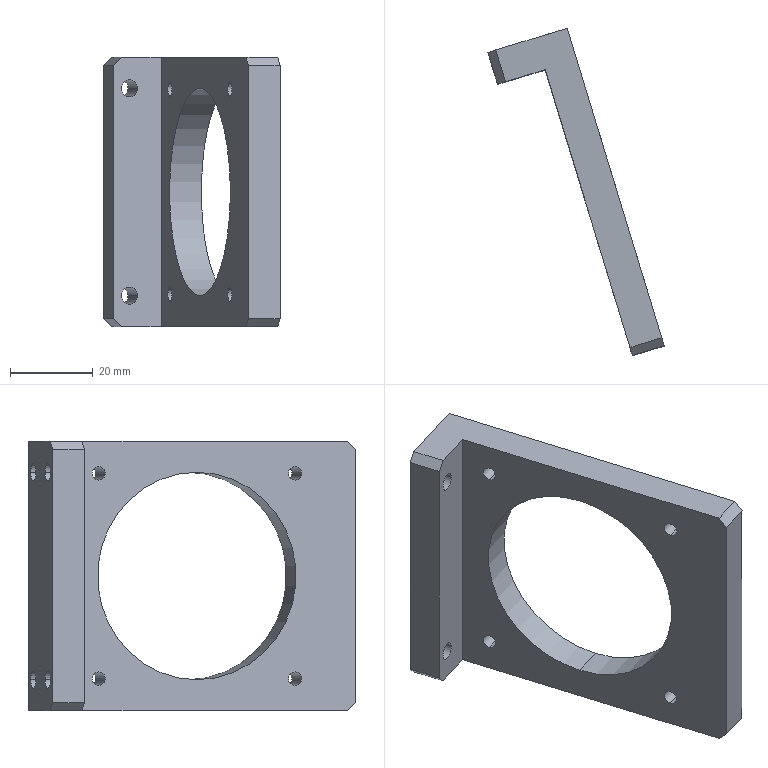Component | SolidWorks | V1ZHXTMotorMountingPlateSB1-1 | 1 solid | 34 faces | box 42.48 x 78.85 x 65 mm | volume 31229 mm3 | cylinder 18 | plane 12 | cone 4 | commonest cylinder face diameters 4.2 x8 3.3 x8 50 x2
STEP:
#1=CARTESIAN_POINT('',(6.593,-7.94,10.049));
#2=VERTEX_POINT('',#1);
#3=CARTESIAN_POINT('',(6.435,-7.988,10.049));
#4=VERTEX_POINT('',#3);
#5=CARTESIAN_POINT('',(6.514,-7.964,10.049));
#6=DIRECTION('',(0.2918,-0.9565,-0.));
#7=DIRECTION('',(-0.9565,-0.2918,-0.));
#8=AXIS2_PLACEMENT_3D('',#5,#6,#7);
#9=CIRCLE('',#8,0.08268);
#10=EDGE_CURVE('',#2,#4,#9,.T.);
#11=ORIENTED_EDGE('',*,*,#10,.T.);
#12=CARTESIAN_POINT('',(6.343,-7.687,10.049));
#13=VERTEX_POINT('',#12);
#14=CARTESIAN_POINT('',(6.343,-7.687,10.049));
#15=DIRECTION('',(-0.2918,0.9565,0.));
#16=VECTOR('',#15,39.37);
#17=LINE('',#14,#16);
#18=EDGE_CURVE('',#4,#13,#17,.T.);
#19=ORIENTED_EDGE('',*,*,#18,.T.);
#20=CARTESIAN_POINT('',(6.502,-7.638,10.049));
#21=VERTEX_POINT('',#20);
#22=CARTESIAN_POINT('',(6.422,-7.662,10.049));
#23=DIRECTION('',(-0.2918,0.9565,0.));
#24=DIRECTION('',(0.9565,0.2918,0.));
#25=AXIS2_PLACEMENT_3D('',#22,#23,#24);
#26=CIRCLE('',#25,0.08268);
#27=EDGE_CURVE('',#13,#21,#26,.T.);
#28=ORIENTED_EDGE('',*,*,#27,.T.);
#29=CARTESIAN_POINT('',(6.502,-7.638,10.049));
#30=DIRECTION('',(-0.2918,0.9565,0.));
#31=VECTOR('',#30,39.37);
#32=LINE('',#29,#31);
#33=EDGE_CURVE('',#2,#21,#32,.T.);
#34=ORIENTED_EDGE('',*,*,#33,.F.);
#35=EDGE_LOOP('',(#11,#19,#28,#34));
#36=FACE_OUTER_BOUND('',#35,.T.);
#37=CARTESIAN_POINT('',(6.422,-7.662,10.049));
#38=DIRECTION('',(-0.2918,0.9565,0.));
#39=DIRECTION('',(0.9565,0.2918,0.));
#40=AXIS2_PLACEMENT_3D('',#37,#38,#39);
#41=CYLINDRICAL_SURFACE('',#40,0.08268);
#42=ADVANCED_FACE('',(#36),#41,.F.);
#43=CARTESIAN_POINT('',(6.593,-7.94,12.017));
#44=VERTEX_POINT('',#43);
#45=CARTESIAN_POINT('',(6.435,-7.988,12.017));
#46=VERTEX_POINT('',#45);
#47=CARTESIAN_POINT('',(6.514,-7.964,12.017));
#48=DIRECTION('',(0.2918,-0.9565,-0.));
#49=DIRECTION('',(-0.9565,-0.2918,-0.));
#50=AXIS2_PLACEMENT_3D('',#47,#48,#49);
#51=CIRCLE('',#50,0.08268);
#52=EDGE_CURVE('',#44,#46,#51,.T.);
#53=ORIENTED_EDGE('',*,*,#52,.T.);
#54=CARTESIAN_POINT('',(6.343,-7.687,12.017));
#55=VERTEX_POINT('',#54);
#56=CARTESIAN_POINT('',(6.343,-7.687,12.017));
#57=DIRECTION('',(-0.2918,0.9565,0.));
#58=VECTOR('',#57,39.37);
#59=LINE('',#56,#58);
#60=EDGE_CURVE('',#46,#55,#59,.T.);
#61=ORIENTED_EDGE('',*,*,#60,.T.);
#62=CARTESIAN_POINT('',(6.502,-7.638,12.017));
#63=VERTEX_POINT('',#62);
#64=CARTESIAN_POINT('',(6.422,-7.662,12.017));
#65=DIRECTION('',(-0.2918,0.9565,0.));
#66=DIRECTION('',(0.9565,0.2918,0.));
#67=AXIS2_PLACEMENT_3D('',#64,#65,#66);
#68=CIRCLE('',#67,0.08268);
#69=EDGE_CURVE('',#55,#63,#68,.T.);
#70=ORIENTED_EDGE('',*,*,#69,.T.);
#71=CARTESIAN_POINT('',(6.502,-7.638,12.017));
#72=DIRECTION('',(-0.2918,0.9565,0.));
#73=VECTOR('',#72,39.37);
#74=LINE('',#71,#73);
#75=EDGE_CURVE('',#44,#63,#74,.T.);
#76=ORIENTED_EDGE('',*,*,#75,.F.);
#77=EDGE_LOOP('',(#53,#61,#70,#76));
#78=FACE_OUTER_BOUND('',#77,.T.);
#79=CARTESIAN_POINT('',(6.422,-7.662,12.017));
#80=DIRECTION('',(-0.2918,0.9565,0.));
#81=DIRECTION('',(0.9565,0.2918,0.));
#82=AXIS2_PLACEMENT_3D('',#79,#80,#81);
#83=CYLINDRICAL_SURFACE('',#82,0.08268);
#84=ADVANCED_FACE('',(#78),#83,.F.);
#85=CARTESIAN_POINT('',(6.933,-8.001,10.049));
#86=VERTEX_POINT('',#85);
#87=CARTESIAN_POINT('',(7.091,-7.952,10.049));
#88=VERTEX_POINT('',#87);
#89=CARTESIAN_POINT('',(7.012,-7.976,10.049));
#90=DIRECTION('',(-0.2918,0.9565,0.));
#91=DIRECTION('',(0.9565,0.2918,0.));
#92=AXIS2_PLACEMENT_3D('',#89,#90,#91);
#93=CIRCLE('',#92,0.08268);
#94=EDGE_CURVE('',#86,#88,#93,.T.);
#95=ORIENTED_EDGE('',*,*,#94,.F.);
#96=CARTESIAN_POINT('',(6.795,-7.549,10.049));
#97=VERTEX_POINT('',#96);
#98=CARTESIAN_POINT('',(6.795,-7.549,10.049));
#99=DIRECTION('',(-0.2918,0.9565,0.));
#100=VECTOR('',#99,39.37);
#101=LINE('',#98,#100);
#102=EDGE_CURVE('',#86,#97,#101,.T.);
#103=ORIENTED_EDGE('',*,*,#102,.T.);
#104=CARTESIAN_POINT('',(6.953,-7.5,10.049));
#105=VERTEX_POINT('',#104);
#106=CARTESIAN_POINT('',(6.874,-7.525,10.049));
#107=DIRECTION('',(-0.2918,0.9565,0.));
#108=DIRECTION('',(0.9565,0.2918,0.));
#109=AXIS2_PLACEMENT_3D('',#106,#107,#108);
#110=CIRCLE('',#109,0.08268);
#111=EDGE_CURVE('',#97,#105,#110,.T.);
#112=ORIENTED_EDGE('',*,*,#111,.T.);
#113=CARTESIAN_POINT('',(6.953,-7.5,10.049));
#114=DIRECTION('',(-0.2918,0.9565,0.));
#115=VECTOR('',#114,39.37);
#116=LINE('',#113,#115);
#117=EDGE_CURVE('',#88,#105,#116,.T.);
#118=ORIENTED_EDGE('',*,*,#117,.F.);
#119=EDGE_LOOP('',(#95,#103,#112,#118));
#120=FACE_OUTER_BOUND('',#119,.T.);
#121=CARTESIAN_POINT('',(6.874,-7.525,10.049));
#122=DIRECTION('',(-0.2918,0.9565,0.));
#123=DIRECTION('',(0.9565,0.2918,0.));
#124=AXIS2_PLACEMENT_3D('',#121,#122,#123);
#125=CYLINDRICAL_SURFACE('',#124,0.08268);
#126=ADVANCED_FACE('',(#120),#125,.F.);
#127=CARTESIAN_POINT('',(7.027,-8.024,10.049));
#128=VERTEX_POINT('',#127);
#129=CARTESIAN_POINT('',(7.091,-7.952,10.049));
#130=DIRECTION('',(0.6696,0.7428,0.));
#131=VECTOR('',#130,39.37);
#132=LINE('',#129,#131);
#133=EDGE_CURVE('',#128,#88,#132,.T.);
#134=ORIENTED_EDGE('',*,*,#133,.F.);
#135=CARTESIAN_POINT('',(6.933,-8.001,10.049));
#136=DIRECTION('',(-0.9702,0.2425,0.));
#137=VECTOR('',#136,39.37);
#138=LINE('',#135,#137);
#139=EDGE_CURVE('',#128,#86,#138,.T.);
#140=ORIENTED_EDGE('',*,*,#139,.T.);
#141=ORIENTED_EDGE('',*,*,#94,.T.);
#142=EDGE_LOOP('',(#134,#140,#141));
#143=FACE_OUTER_BOUND('',#142,.T.);
#144=CARTESIAN_POINT('',(7.012,-7.976,10.049));
#145=DIRECTION('',(-0.2918,0.9565,0.));
#146=DIRECTION('',(0.9565,0.2918,0.));
#147=AXIS2_PLACEMENT_3D('',#144,#145,#146);
#148=CONICAL_SURFACE('',#147,0.08268,1.03);
#149=ADVANCED_FACE('',(#143),#148,.F.);
#150=CARTESIAN_POINT('',(6.933,-8.001,12.017));
#151=VERTEX_POINT('',#150);
#152=CARTESIAN_POINT('',(7.091,-7.952,12.017));
#153=VERTEX_POINT('',#152);
#154=CARTESIAN_POINT('',(7.012,-7.976,12.017));
#155=DIRECTION('',(-0.2918,0.9565,0.));
#156=DIRECTION('',(0.9565,0.2918,0.));
#157=AXIS2_PLACEMENT_3D('',#154,#155,#156);
#158=CIRCLE('',#157,0.08268);
#159=EDGE_CURVE('',#151,#153,#158,.T.);
#160=ORIENTED_EDGE('',*,*,#159,.F.);
#161=CARTESIAN_POINT('',(6.795,-7.549,12.017));
#162=VERTEX_POINT('',#161);
#163=CARTESIAN_POINT('',(6.795,-7.549,12.017));
#164=DIRECTION('',(-0.2918,0.9565,0.));
#165=VECTOR('',#164,39.37);
#166=LINE('',#163,#165);
#167=EDGE_CURVE('',#151,#162,#166,.T.);
#168=ORIENTED_EDGE('',*,*,#167,.T.);
#169=CARTESIAN_POINT('',(6.953,-7.5,12.017));
#170=VERTEX_POINT('',#169);
#171=CARTESIAN_POINT('',(6.874,-7.525,12.017));
#172=DIRECTION('',(-0.2918,0.9565,0.));
#173=DIRECTION('',(0.9565,0.2918,0.));
#174=AXIS2_PLACEMENT_3D('',#171,#172,#173);
#175=CIRCLE('',#174,0.08268);
#176=EDGE_CURVE('',#162,#170,#175,.T.);
#177=ORIENTED_EDGE('',*,*,#176,.T.);
#178=CARTESIAN_POINT('',(6.953,-7.5,12.017));
#179=DIRECTION('',(-0.2918,0.9565,0.));
#180=VECTOR('',#179,39.37);
#181=LINE('',#178,#180);
#182=EDGE_CURVE('',#153,#170,#181,.T.);
#183=ORIENTED_EDGE('',*,*,#182,.F.);
#184=EDGE_LOOP('',(#160,#168,#177,#183));
#185=FACE_OUTER_BOUND('',#184,.T.);
#186=CARTESIAN_POINT('',(6.874,-7.525,12.017));
#187=DIRECTION('',(-0.2918,0.9565,0.));
#188=DIRECTION('',(0.9565,0.2918,0.));
#189=AXIS2_PLACEMENT_3D('',#186,#187,#188);
#190=CYLINDRICAL_SURFACE('',#189,0.08268);
#191=ADVANCED_FACE('',(#185),#190,.F.);
#192=CARTESIAN_POINT('',(7.027,-8.024,12.017));
#193=VERTEX_POINT('',#192);
#194=CARTESIAN_POINT('',(7.091,-7.952,12.017));
#195=DIRECTION('',(0.6696,0.7428,0.));
#196=VECTOR('',#195,39.37);
#197=LINE('',#194,#196);
#198=EDGE_CURVE('',#193,#153,#197,.T.);
#199=ORIENTED_EDGE('',*,*,#198,.F.);
#200=CARTESIAN_POINT('',(6.933,-8.001,12.017));
#201=DIRECTION('',(-0.9702,0.2425,0.));
#202=VECTOR('',#201,39.37);
#203=LINE('',#200,#202);
#204=EDGE_CURVE('',#193,#151,#203,.T.);
#205=ORIENTED_EDGE('',*,*,#204,.T.);
#206=ORIENTED_EDGE('',*,*,#159,.T.);
#207=EDGE_LOOP('',(#199,#205,#206));
#208=FACE_OUTER_BOUND('',#207,.T.);
#209=CARTESIAN_POINT('',(7.012,-7.976,12.017));
#210=DIRECTION('',(-0.2918,0.9565,0.));
#211=DIRECTION('',(0.9565,0.2918,0.));
#212=AXIS2_PLACEMENT_3D('',#209,#210,#211);
#213=CONICAL_SURFACE('',#212,0.08268,1.03);
#214=ADVANCED_FACE('',(#208),#213,.F.);
#215=CARTESIAN_POINT('',(7.2,-8.053,10.124));
#216=VERTEX_POINT('',#215);
#217=CARTESIAN_POINT('',(7.2,-8.053,9.994));
#218=VERTEX_POINT('',#217);
#219=CARTESIAN_POINT('',(7.2,-8.053,10.059));
#220=DIRECTION('',(-0.9565,-0.2918,-0.));
#221=DIRECTION('',(0.,0.,-1.));
#222=AXIS2_PLACEMENT_3D('',#219,#220,#221);
#223=CIRCLE('',#222,0.06496);
#224=EDGE_CURVE('',#216,#218,#223,.T.);
#225=ORIENTED_EDGE('',*,*,#224,.F.);
#226=CARTESIAN_POINT('',(6.899,-8.145,10.124));
#227=VERTEX_POINT('',#226);
#228=CARTESIAN_POINT('',(6.899,-8.145,10.124));
#229=DIRECTION('',(-0.9565,-0.2918,-0.));
#230=VECTOR('',#229,39.37);
#231=LINE('',#228,#230);
#232=EDGE_CURVE('',#216,#227,#231,.T.);
#233=ORIENTED_EDGE('',*,*,#232,.T.);
#234=CARTESIAN_POINT('',(6.899,-8.145,9.994));
#235=VERTEX_POINT('',#234);
#236=CARTESIAN_POINT('',(6.899,-8.145,10.059));
#237=DIRECTION('',(-0.9565,-0.2918,-0.));
#238=DIRECTION('',(0.,0.,-1.));
#239=AXIS2_PLACEMENT_3D('',#236,#237,#238);
#240=CIRCLE('',#239,0.06496);
#241=EDGE_CURVE('',#227,#235,#240,.T.);
#242=ORIENTED_EDGE('',*,*,#241,.T.);
#243=CARTESIAN_POINT('',(6.899,-8.145,9.994));
#244=DIRECTION('',(-0.9565,-0.2918,-0.));
#245=VECTOR('',#244,39.37);
#246=LINE('',#243,#245);
#247=EDGE_CURVE('',#218,#235,#246,.T.);
#248=ORIENTED_EDGE('',*,*,#247,.F.);
#249=EDGE_LOOP('',(#225,#233,#242,#248));
#250=FACE_OUTER_BOUND('',#249,.T.);
#251=CARTESIAN_POINT('',(6.899,-8.145,10.059));
#252=DIRECTION('',(-0.9565,-0.2918,-0.));
#253=DIRECTION('',(0.,0.,-1.));
#254=AXIS2_PLACEMENT_3D('',#251,#252,#253);
#255=CYLINDRICAL_SURFACE('',#254,0.06496);
#256=ADVANCED_FACE('',(#250),#255,.F.);
#257=CARTESIAN_POINT('',(7.2,-8.053,12.072));
#258=VERTEX_POINT('',#257);
#259=CARTESIAN_POINT('',(7.2,-8.053,11.942));
#260=VERTEX_POINT('',#259);
#261=CARTESIAN_POINT('',(7.2,-8.053,12.007));
#262=DIRECTION('',(-0.9565,-0.2918,-0.));
#263=DIRECTION('',(0.,0.,-1.));
#264=AXIS2_PLACEMENT_3D('',#261,#262,#263);
#265=CIRCLE('',#264,0.06496);
#266=EDGE_CURVE('',#258,#260,#265,.T.);
#267=ORIENTED_EDGE('',*,*,#266,.F.);
#268=CARTESIAN_POINT('',(6.899,-8.145,12.072));
#269=VERTEX_POINT('',#268);
#270=CARTESIAN_POINT('',(6.899,-8.145,12.072));
#271=DIRECTION('',(-0.9565,-0.2918,-0.));
#272=VECTOR('',#271,39.37);
#273=LINE('',#270,#272);
#274=EDGE_CURVE('',#258,#269,#273,.T.);
#275=ORIENTED_EDGE('',*,*,#274,.T.);
#276=CARTESIAN_POINT('',(6.899,-8.145,11.942));
#277=VERTEX_POINT('',#276);
#278=CARTESIAN_POINT('',(6.899,-8.145,12.007));
#279=DIRECTION('',(-0.9565,-0.2918,-0.));
#280=DIRECTION('',(0.,0.,-1.));
#281=AXIS2_PLACEMENT_3D('',#278,#279,#280);
#282=CIRCLE('',#281,0.06496);
#283=EDGE_CURVE('',#269,#277,#282,.T.);
#284=ORIENTED_EDGE('',*,*,#283,.T.);
#285=CARTESIAN_POINT('',(6.899,-8.145,11.942));
#286=DIRECTION('',(-0.9565,-0.2918,-0.));
#287=VECTOR('',#286,39.37);
#288=LINE('',#285,#287);
#289=EDGE_CURVE('',#260,#277,#288,.T.);
#290=ORIENTED_EDGE('',*,*,#289,.F.);
#291=EDGE_LOOP('',(#267,#275,#284,#290));
#292=FACE_OUTER_BOUND('',#291,.T.);
#293=CARTESIAN_POINT('',(6.899,-8.145,12.007));
#294=DIRECTION('',(-0.9565,-0.2918,-0.));
#295=DIRECTION('',(0.,0.,-1.));
#296=AXIS2_PLACEMENT_3D('',#293,#294,#295);
#297=CYLINDRICAL_SURFACE('',#296,0.06496);
#298=ADVANCED_FACE('',(#292),#297,.F.);
#299=CARTESIAN_POINT('',(7.769,-9.917,12.072));
#300=VERTEX_POINT('',#299);
#301=CARTESIAN_POINT('',(7.769,-9.917,11.942));
#302=VERTEX_POINT('',#301);
#303=CARTESIAN_POINT('',(7.769,-9.917,12.007));
#304=DIRECTION('',(-0.9565,-0.2918,-0.));
#305=DIRECTION('',(0.,0.,-1.));
#306=AXIS2_PLACEMENT_3D('',#303,#304,#305);
#307=CIRCLE('',#306,0.06496);
#308=EDGE_CURVE('',#300,#302,#307,.T.);
#309=ORIENTED_EDGE('',*,*,#308,.F.);
#310=CARTESIAN_POINT('',(7.468,-10.009,12.072));
#311=VERTEX_POINT('',#310);
#312=CARTESIAN_POINT('',(7.468,-10.009,12.072));
#313=DIRECTION('',(-0.9565,-0.2918,-0.));
#314=VECTOR('',#313,39.37);
#315=LINE('',#312,#314);
#316=EDGE_CURVE('',#300,#311,#315,.T.);
#317=ORIENTED_EDGE('',*,*,#316,.T.);
#318=CARTESIAN_POINT('',(7.468,-10.009,11.942));
#319=VERTEX_POINT('',#318);
#320=CARTESIAN_POINT('',(7.468,-10.009,12.007));
#321=DIRECTION('',(-0.9565,-0.2918,-0.));
#322=DIRECTION('',(0.,0.,-1.));
#323=AXIS2_PLACEMENT_3D('',#320,#321,#322);
#324=CIRCLE('',#323,0.06496);
#325=EDGE_CURVE('',#311,#319,#324,.T.);
#326=ORIENTED_EDGE('',*,*,#325,.T.);
#327=CARTESIAN_POINT('',(7.468,-10.009,11.942));
#328=DIRECTION('',(-0.9565,-0.2918,-0.));
#329=VECTOR('',#328,39.37);
#330=LINE('',#327,#329);
#331=EDGE_CURVE('',#302,#319,#330,.T.);
#332=ORIENTED_EDGE('',*,*,#331,.F.);
#333=EDGE_LOOP('',(#309,#317,#326,#332));
#334=FACE_OUTER_BOUND('',#333,.T.);
#335=CARTESIAN_POINT('',(7.468,-10.009,12.007));
#336=DIRECTION('',(-0.9565,-0.2918,-0.));
#337=DIRECTION('',(0.,0.,-1.));
#338=AXIS2_PLACEMENT_3D('',#335,#336,#337);
#339=CYLINDRICAL_SURFACE('',#338,0.06496);
#340=ADVANCED_FACE('',(#334),#339,.F.);
#341=CARTESIAN_POINT('',(7.769,-9.917,10.124));
#342=VERTEX_POINT('',#341);
#343=CARTESIAN_POINT('',(7.769,-9.917,9.994));
#344=VERTEX_POINT('',#343);
#345=CARTESIAN_POINT('',(7.769,-9.917,10.059));
#346=DIRECTION('',(-0.9565,-0.2918,-0.));
#347=DIRECTION('',(0.,0.,-1.));
#348=AXIS2_PLACEMENT_3D('',#345,#346,#347);
#349=CIRCLE('',#348,0.06496);
#350=EDGE_CURVE('',#342,#344,#349,.T.);
#351=ORIENTED_EDGE('',*,*,#350,.F.);
#352=CARTESIAN_POINT('',(7.468,-10.009,10.124));
#353=VERTEX_POINT('',#352);
#354=CARTESIAN_POINT('',(7.468,-10.009,10.124));
#355=DIRECTION('',(-0.9565,-0.2918,-0.));
#356=VECTOR('',#355,39.37);
#357=LINE('',#354,#356);
#358=EDGE_CURVE('',#342,#353,#357,.T.);
#359=ORIENTED_EDGE('',*,*,#358,.T.);
#360=CARTESIAN_POINT('',(7.468,-10.009,9.994));
#361=VERTEX_POINT('',#360);
#362=CARTESIAN_POINT('',(7.468,-10.009,10.059));
#363=DIRECTION('',(-0.9565,-0.2918,-0.));
#364=DIRECTION('',(0.,0.,-1.));
#365=AXIS2_PLACEMENT_3D('',#362,#363,#364);
#366=CIRCLE('',#365,0.06496);
#367=EDGE_CURVE('',#353,#361,#366,.T.);
#368=ORIENTED_EDGE('',*,*,#367,.T.);
#369=CARTESIAN_POINT('',(7.468,-10.009,9.994));
#370=DIRECTION('',(-0.9565,-0.2918,-0.));
#371=VECTOR('',#370,39.37);
#372=LINE('',#369,#371);
#373=EDGE_CURVE('',#344,#361,#372,.T.);
#374=ORIENTED_EDGE('',*,*,#373,.F.);
#375=EDGE_LOOP('',(#351,#359,#368,#374));
#376=FACE_OUTER_BOUND('',#375,.T.);
#377=CARTESIAN_POINT('',(7.468,-10.009,10.059));
#378=DIRECTION('',(-0.9565,-0.2918,-0.));
#379=DIRECTION('',(0.,0.,-1.));
#380=AXIS2_PLACEMENT_3D('',#377,#378,#379);
#381=CYLINDRICAL_SURFACE('',#380,0.06496);
#382=ADVANCED_FACE('',(#376),#381,.F.);
#383=CARTESIAN_POINT('',(7.485,-8.985,12.017));
#384=VERTEX_POINT('',#383);
#385=CARTESIAN_POINT('',(7.485,-8.985,10.049));
#386=VERTEX_POINT('',#385);
#387=CARTESIAN_POINT('',(7.485,-8.985,11.033));
#388=DIRECTION('',(-0.9565,-0.2918,-0.));
#389=DIRECTION('',(0.,0.,-1.));
#390=AXIS2_PLACEMENT_3D('',#387,#388,#389);
#391=CIRCLE('',#390,0.9843);
#392=EDGE_CURVE('',#384,#386,#391,.T.);
#393=ORIENTED_EDGE('',*,*,#392,.F.);
#394=CARTESIAN_POINT('',(7.183,-9.077,12.017));
#395=VERTEX_POINT('',#394);
#396=CARTESIAN_POINT('',(7.485,-8.985,12.017));
#397=DIRECTION('',(-0.9565,-0.2918,-0.));
#398=VECTOR('',#397,39.37);
#399=LINE('',#396,#398);
#400=EDGE_CURVE('',#384,#395,#399,.T.);
#401=ORIENTED_EDGE('',*,*,#400,.T.);
#402=CARTESIAN_POINT('',(7.183,-9.077,10.049));
#403=VERTEX_POINT('',#402);
#404=CARTESIAN_POINT('',(7.183,-9.077,11.033));
#405=DIRECTION('',(-0.9565,-0.2918,-0.));
#406=DIRECTION('',(0.,0.,-1.));
#407=AXIS2_PLACEMENT_3D('',#404,#405,#406);
#408=CIRCLE('',#407,0.9843);
#409=EDGE_CURVE('',#395,#403,#408,.T.);
#410=ORIENTED_EDGE('',*,*,#409,.T.);
#411=CARTESIAN_POINT('',(7.485,-8.985,10.049));
#412=DIRECTION('',(-0.9565,-0.2918,-0.));
#413=VECTOR('',#412,39.37);
#414=LINE('',#411,#413);
#415=EDGE_CURVE('',#386,#403,#414,.T.);
#416=ORIENTED_EDGE('',*,*,#415,.F.);
#417=EDGE_LOOP('',(#393,#401,#410,#416));
#418=FACE_OUTER_BOUND('',#417,.T.);
#419=CARTESIAN_POINT('',(7.485,-8.985,11.033));
#420=DIRECTION('',(-0.9565,-0.2918,-0.));
#421=DIRECTION('',(0.,0.,-1.));
#422=AXIS2_PLACEMENT_3D('',#419,#420,#421);
#423=CYLINDRICAL_SURFACE('',#422,0.9843);
#424=ADVANCED_FACE('',(#418),#423,.F.);
#425=CARTESIAN_POINT('',(7.944,-10.491,9.832));
#426=VERTEX_POINT('',#425);
#427=CARTESIAN_POINT('',(7.921,-10.416,9.754));
#428=VERTEX_POINT('',#427);
#429=CARTESIAN_POINT('',(7.89,-10.312,9.645));
#430=DIRECTION('',(-0.2064,0.6763,-0.7071));
#431=VECTOR('',#430,39.37);
#432=LINE('',#429,#431);
#433=EDGE_CURVE('',#426,#428,#432,.T.);
#434=ORIENTED_EDGE('',*,*,#433,.T.);
#435=CARTESIAN_POINT('',(7.025,-7.479,9.754));
#436=VERTEX_POINT('',#435);
#437=CARTESIAN_POINT('',(7.025,-7.479,9.754));
#438=DIRECTION('',(0.2918,-0.9565,-0.));
#439=VECTOR('',#438,39.37);
#440=LINE('',#437,#439);
#441=EDGE_CURVE('',#436,#428,#440,.T.);
#442=ORIENTED_EDGE('',*,*,#441,.F.);
#443=CARTESIAN_POINT('',(7.025,-7.479,12.313));
#444=VERTEX_POINT('',#443);
#445=CARTESIAN_POINT('',(7.025,-7.479,12.313));
#446=DIRECTION('',(0.,0.,-1.));
#447=VECTOR('',#446,39.37);
#448=LINE('',#445,#447);
#449=EDGE_CURVE('',#444,#436,#448,.T.);
#450=ORIENTED_EDGE('',*,*,#449,.F.);
#451=CARTESIAN_POINT('',(7.921,-10.416,12.313));
#452=VERTEX_POINT('',#451);
#453=CARTESIAN_POINT('',(7.025,-7.479,12.313));
#454=DIRECTION('',(-0.2918,0.9565,0.));
#455=VECTOR('',#454,39.37);
#456=LINE('',#453,#455);
#457=EDGE_CURVE('',#452,#444,#456,.T.);
#458=ORIENTED_EDGE('',*,*,#457,.F.);
#459=CARTESIAN_POINT('',(7.944,-10.491,12.234));
#460=VERTEX_POINT('',#459);
#461=CARTESIAN_POINT('',(7.89,-10.312,12.421));
#462=DIRECTION('',(0.2064,-0.6763,-0.7071));
#463=VECTOR('',#462,39.37);
#464=LINE('',#461,#463);
#465=EDGE_CURVE('',#452,#460,#464,.T.);
#466=ORIENTED_EDGE('',*,*,#465,.T.);
#467=CARTESIAN_POINT('',(7.944,-10.491,12.313));
#468=DIRECTION('',(-0.,-0.,1.));
#469=VECTOR('',#468,39.37);
#470=LINE('',#467,#469);
#471=EDGE_CURVE('',#426,#460,#470,.T.);
#472=ORIENTED_EDGE('',*,*,#471,.F.);
#473=EDGE_LOOP('',(#434,#442,#450,#458,#466,#472));
#474=FACE_OUTER_BOUND('',#473,.T.);
#475=CARTESIAN_POINT('',(7.2,-8.053,10.059));
#476=DIRECTION('',(-0.9565,-0.2918,-0.));
#477=DIRECTION('',(0.,0.,-1.));
#478=AXIS2_PLACEMENT_3D('',#475,#476,#477);
#479=CIRCLE('',#478,0.06496);
#480=EDGE_CURVE('',#218,#216,#479,.T.);
#481=ORIENTED_EDGE('',*,*,#480,.T.);
#482=ORIENTED_EDGE('',*,*,#224,.T.);
#483=EDGE_LOOP('',(#481,#482));
#484=FACE_BOUND('',#483,.T.);
#485=CARTESIAN_POINT('',(7.485,-8.985,11.033));
#486=DIRECTION('',(-0.9565,-0.2918,-0.));
#487=DIRECTION('',(0.,0.,-1.));
#488=AXIS2_PLACEMENT_3D('',#485,#486,#487);
#489=CIRCLE('',#488,0.9843);
#490=EDGE_CURVE('',#386,#384,#489,.T.);
#491=ORIENTED_EDGE('',*,*,#490,.T.);
#492=ORIENTED_EDGE('',*,*,#392,.T.);
#493=EDGE_LOOP('',(#491,#492));
#494=FACE_BOUND('',#493,.T.);
#495=CARTESIAN_POINT('',(7.769,-9.917,10.059));
#496=DIRECTION('',(-0.9565,-0.2918,-0.));
#497=DIRECTION('',(0.,0.,-1.));
#498=AXIS2_PLACEMENT_3D('',#495,#496,#497);
#499=CIRCLE('',#498,0.06496);
#500=EDGE_CURVE('',#344,#342,#499,.T.);
#501=ORIENTED_EDGE('',*,*,#500,.T.);
#502=ORIENTED_EDGE('',*,*,#350,.T.);
#503=EDGE_LOOP('',(#501,#502));
#504=FACE_BOUND('',#503,.T.);
#505=CARTESIAN_POINT('',(7.769,-9.917,12.007));
#506=DIRECTION('',(-0.9565,-0.2918,-0.));
#507=DIRECTION('',(0.,0.,-1.));
#508=AXIS2_PLACEMENT_3D('',#505,#506,#507);
#509=CIRCLE('',#508,0.06496);
#510=EDGE_CURVE('',#302,#300,#509,.T.);
#511=ORIENTED_EDGE('',*,*,#510,.T.);
#512=ORIENTED_EDGE('',*,*,#308,.T.);
#513=EDGE_LOOP('',(#511,#512));
#514=FACE_BOUND('',#513,.T.);
#515=CARTESIAN_POINT('',(7.2,-8.053,12.007));
#516=DIRECTION('',(-0.9565,-0.2918,-0.));
#517=DIRECTION('',(0.,0.,-1.));
#518=AXIS2_PLACEMENT_3D('',#515,#516,#517);
#519=CIRCLE('',#518,0.06496);
#520=EDGE_CURVE('',#260,#258,#519,.T.);
#521=ORIENTED_EDGE('',*,*,#520,.T.);
#522=ORIENTED_EDGE('',*,*,#266,.T.);
#523=EDGE_LOOP('',(#521,#522));
#524=FACE_BOUND('',#523,.T.);
#525=CARTESIAN_POINT('',(7.485,-8.985,11.033));
#526=DIRECTION('',(0.9565,0.2918,0.));
#527=DIRECTION('',(-0.,-0.,1.));
#528=AXIS2_PLACEMENT_3D('',#525,#526,#527);
#529=PLANE('',#528);
#530=ADVANCED_FACE('',(#474,#484,#494,#504,#514,#524),#529,.T.);
#531=CARTESIAN_POINT('',(6.439,-7.987,9.754));
#532=VERTEX_POINT('',#531);
#533=CARTESIAN_POINT('',(6.816,-7.872,9.754));
#534=VERTEX_POINT('',#533);
#535=CARTESIAN_POINT('',(6.364,-8.01,9.754));
#536=DIRECTION('',(0.9565,0.2918,0.));
#537=VECTOR('',#536,39.37);
#538=LINE('',#535,#537);
#539=EDGE_CURVE('',#532,#534,#538,.T.);
#540=ORIENTED_EDGE('',*,*,#539,.F.);
#541=CARTESIAN_POINT('',(6.347,-7.685,9.754));
#542=VERTEX_POINT('',#541);
#543=CARTESIAN_POINT('',(6.347,-7.685,9.754));
#544=DIRECTION('',(-0.2918,0.9565,0.));
#545=VECTOR('',#544,39.37);
#546=LINE('',#543,#545);
#547=EDGE_CURVE('',#532,#542,#546,.T.);
#548=ORIENTED_EDGE('',*,*,#547,.T.);
#549=CARTESIAN_POINT('',(6.724,-7.571,9.754));
#550=DIRECTION('',(0.9565,0.2918,0.));
#551=VECTOR('',#550,39.37);
#552=LINE('',#549,#551);
#553=EDGE_CURVE('',#542,#436,#552,.T.);
#554=ORIENTED_EDGE('',*,*,#553,.T.);
#555=ORIENTED_EDGE('',*,*,#441,.T.);
#556=CARTESIAN_POINT('',(7.62,-10.508,9.754));
#557=VERTEX_POINT('',#556);
#558=CARTESIAN_POINT('',(7.62,-10.508,9.754));
#559=DIRECTION('',(-0.9565,-0.2918,-0.));
#560=VECTOR('',#559,39.37);
#561=LINE('',#558,#560);
#562=EDGE_CURVE('',#428,#557,#561,.T.);
#563=ORIENTED_EDGE('',*,*,#562,.T.);
#564=CARTESIAN_POINT('',(6.724,-7.571,9.754));
#565=DIRECTION('',(0.2918,-0.9565,-0.));
#566=VECTOR('',#565,39.37);
#567=LINE('',#564,#566);
#568=EDGE_CURVE('',#534,#557,#567,.T.);
#569=ORIENTED_EDGE('',*,*,#568,.F.);
#570=EDGE_LOOP('',(#540,#548,#554,#555,#563,#569));
#571=FACE_OUTER_BOUND('',#570,.T.);
#572=CARTESIAN_POINT('',(6.724,-7.571,9.754));
#573=DIRECTION('',(-0.,-0.,1.));
#574=DIRECTION('',(-0.9565,-0.2918,-0.));
#575=AXIS2_PLACEMENT_3D('',#572,#573,#574);
#576=PLANE('',#575);
#577=ADVANCED_FACE('',(#571),#576,.F.);
#578=ORIENTED_EDGE('',*,*,#471,.T.);
#579=CARTESIAN_POINT('',(7.643,-10.583,12.234));
#580=VERTEX_POINT('',#579);
#581=CARTESIAN_POINT('',(7.643,-10.583,12.234));
#582=DIRECTION('',(-0.9565,-0.2918,-0.));
#583=VECTOR('',#582,39.37);
#584=LINE('',#581,#583);
#585=EDGE_CURVE('',#460,#580,#584,.T.);
#586=ORIENTED_EDGE('',*,*,#585,.T.);
#587=CARTESIAN_POINT('',(7.643,-10.583,9.832));
#588=VERTEX_POINT('',#587);
#589=CARTESIAN_POINT('',(7.643,-10.583,12.313));
#590=DIRECTION('',(-0.,-0.,1.));
#591=VECTOR('',#590,39.37);
#592=LINE('',#589,#591);
#593=EDGE_CURVE('',#588,#580,#592,.T.);
#594=ORIENTED_EDGE('',*,*,#593,.F.);
#595=CARTESIAN_POINT('',(7.643,-10.583,9.832));
#596=DIRECTION('',(0.9565,0.2918,0.));
#597=VECTOR('',#596,39.37);
#598=LINE('',#595,#597);
#599=EDGE_CURVE('',#588,#426,#598,.T.);
#600=ORIENTED_EDGE('',*,*,#599,.T.);
#601=EDGE_LOOP('',(#578,#586,#594,#600));
#602=FACE_OUTER_BOUND('',#601,.T.);
#603=CARTESIAN_POINT('',(7.643,-10.583,12.313));
#604=DIRECTION('',(-0.2918,0.9565,0.));
#605=DIRECTION('',(0.9565,0.2918,0.));
#606=AXIS2_PLACEMENT_3D('',#603,#604,#605);
#607=PLANE('',#606);
#608=ADVANCED_FACE('',(#602),#607,.F.);
#609=CARTESIAN_POINT('',(6.347,-7.685,12.313));
#610=VERTEX_POINT('',#609);
#611=CARTESIAN_POINT('',(6.724,-7.571,12.313));
#612=DIRECTION('',(0.9565,0.2918,0.));
#613=VECTOR('',#612,39.37);
#614=LINE('',#611,#613);
#615=EDGE_CURVE('',#610,#444,#614,.T.);
#616=ORIENTED_EDGE('',*,*,#615,.F.);
#617=CARTESIAN_POINT('',(6.439,-7.987,12.313));
#618=VERTEX_POINT('',#617);
#619=CARTESIAN_POINT('',(6.439,-7.987,12.313));
#620=DIRECTION('',(0.2918,-0.9565,-0.));
#621=VECTOR('',#620,39.37);
#622=LINE('',#619,#621);
#623=EDGE_CURVE('',#610,#618,#622,.T.);
#624=ORIENTED_EDGE('',*,*,#623,.T.);
#625=CARTESIAN_POINT('',(6.816,-7.872,12.313));
#626=VERTEX_POINT('',#625);
#627=CARTESIAN_POINT('',(6.364,-8.01,12.313));
#628=DIRECTION('',(0.9565,0.2918,0.));
#629=VECTOR('',#628,39.37);
#630=LINE('',#627,#629);
#631=EDGE_CURVE('',#618,#626,#630,.T.);
#632=ORIENTED_EDGE('',*,*,#631,.T.);
#633=CARTESIAN_POINT('',(7.62,-10.508,12.313));
#634=VERTEX_POINT('',#633);
#635=CARTESIAN_POINT('',(6.724,-7.571,12.313));
#636=DIRECTION('',(-0.2918,0.9565,0.));
#637=VECTOR('',#636,39.37);
#638=LINE('',#635,#637);
#639=EDGE_CURVE('',#634,#626,#638,.T.);
#640=ORIENTED_EDGE('',*,*,#639,.F.);
#641=CARTESIAN_POINT('',(7.62,-10.508,12.313));
#642=DIRECTION('',(0.9565,0.2918,0.));
#643=VECTOR('',#642,39.37);
#644=LINE('',#641,#643);
#645=EDGE_CURVE('',#634,#452,#644,.T.);
#646=ORIENTED_EDGE('',*,*,#645,.T.);
#647=ORIENTED_EDGE('',*,*,#457,.T.);
#648=EDGE_LOOP('',(#616,#624,#632,#640,#646,#647));
#649=FACE_OUTER_BOUND('',#648,.T.);
#650=CARTESIAN_POINT('',(6.724,-7.571,12.313));
#651=DIRECTION('',(0.,0.,-1.));
#652=DIRECTION('',(0.9565,0.2918,0.));
#653=AXIS2_PLACEMENT_3D('',#650,#651,#652);
#654=PLANE('',#653);
#655=ADVANCED_FACE('',(#649),#654,.F.);
#656=CARTESIAN_POINT('',(6.422,-7.662,10.049));
#657=DIRECTION('',(-0.2918,0.9565,0.));
#658=DIRECTION('',(0.9565,0.2918,0.));
#659=AXIS2_PLACEMENT_3D('',#656,#657,#658);
#660=CIRCLE('',#659,0.08268);
#661=EDGE_CURVE('',#21,#13,#660,.T.);
#662=ORIENTED_EDGE('',*,*,#661,.F.);
#663=ORIENTED_EDGE('',*,*,#27,.F.);
#664=EDGE_LOOP('',(#662,#663));
#665=FACE_BOUND('',#664,.T.);
#666=CARTESIAN_POINT('',(6.422,-7.662,12.017));
#667=DIRECTION('',(-0.2918,0.9565,0.));
#668=DIRECTION('',(0.9565,0.2918,0.));
#669=AXIS2_PLACEMENT_3D('',#666,#667,#668);
#670=CIRCLE('',#669,0.08268);
#671=EDGE_CURVE('',#63,#55,#670,.T.);
#672=ORIENTED_EDGE('',*,*,#671,.F.);
#673=ORIENTED_EDGE('',*,*,#69,.F.);
#674=EDGE_LOOP('',(#672,#673));
#675=FACE_BOUND('',#674,.T.);
#676=CARTESIAN_POINT('',(6.874,-7.525,10.049));
#677=DIRECTION('',(-0.2918,0.9565,0.));
#678=DIRECTION('',(0.9565,0.2918,0.));
#679=AXIS2_PLACEMENT_3D('',#676,#677,#678);
#680=CIRCLE('',#679,0.08268);
#681=EDGE_CURVE('',#105,#97,#680,.T.);
#682=ORIENTED_EDGE('',*,*,#681,.F.);
#683=ORIENTED_EDGE('',*,*,#111,.F.);
#684=EDGE_LOOP('',(#682,#683));
#685=FACE_BOUND('',#684,.T.);
#686=CARTESIAN_POINT('',(6.874,-7.525,12.017));
#687=DIRECTION('',(-0.2918,0.9565,0.));
#688=DIRECTION('',(0.9565,0.2918,0.));
#689=AXIS2_PLACEMENT_3D('',#686,#687,#688);
#690=CIRCLE('',#689,0.08268);
#691=EDGE_CURVE('',#170,#162,#690,.T.);
#692=ORIENTED_EDGE('',*,*,#691,.F.);
#693=ORIENTED_EDGE('',*,*,#176,.F.);
#694=EDGE_LOOP('',(#692,#693));
#695=FACE_BOUND('',#694,.T.);
#696=CARTESIAN_POINT('',(6.272,-7.708,9.832));
#697=VERTEX_POINT('',#696);
#698=CARTESIAN_POINT('',(6.272,-7.708,12.234));
#699=VERTEX_POINT('',#698);
#700=CARTESIAN_POINT('',(6.272,-7.708,9.754));
#701=DIRECTION('',(-0.,-0.,1.));
#702=VECTOR('',#701,39.37);
#703=LINE('',#700,#702);
#704=EDGE_CURVE('',#697,#699,#703,.T.);
#705=ORIENTED_EDGE('',*,*,#704,.T.);
#706=CARTESIAN_POINT('',(6.347,-7.685,12.313));
#707=DIRECTION('',(0.6763,0.2064,0.7071));
#708=VECTOR('',#707,39.37);
#709=LINE('',#706,#708);
#710=EDGE_CURVE('',#699,#610,#709,.T.);
#711=ORIENTED_EDGE('',*,*,#710,.T.);
#712=ORIENTED_EDGE('',*,*,#615,.T.);
#713=ORIENTED_EDGE('',*,*,#449,.T.);
#714=ORIENTED_EDGE('',*,*,#553,.F.);
#715=CARTESIAN_POINT('',(6.347,-7.685,9.754));
#716=DIRECTION('',(-0.6763,-0.2064,0.7071));
#717=VECTOR('',#716,39.37);
#718=LINE('',#715,#717);
#719=EDGE_CURVE('',#542,#697,#718,.T.);
#720=ORIENTED_EDGE('',*,*,#719,.T.);
#721=EDGE_LOOP('',(#705,#711,#712,#713,#714,#720));
#722=FACE_OUTER_BOUND('',#721,.T.);
#723=CARTESIAN_POINT('',(6.724,-7.571,12.313));
#724=DIRECTION('',(0.2918,-0.9565,-0.));
#725=DIRECTION('',(-0.9565,-0.2918,-0.));
#726=AXIS2_PLACEMENT_3D('',#723,#724,#725);
#727=PLANE('',#726);
#728=ADVANCED_FACE('',(#665,#675,#685,#695,#722),#727,.F.);
#729=CARTESIAN_POINT('',(6.899,-8.145,10.059));
#730=DIRECTION('',(-0.9565,-0.2918,-0.));
#731=DIRECTION('',(0.,0.,-1.));
#732=AXIS2_PLACEMENT_3D('',#729,#730,#731);
#733=CIRCLE('',#732,0.06496);
#734=EDGE_CURVE('',#235,#227,#733,.T.);
#735=ORIENTED_EDGE('',*,*,#734,.F.);
#736=ORIENTED_EDGE('',*,*,#241,.F.);
#737=EDGE_LOOP('',(#735,#736));
#738=FACE_BOUND('',#737,.T.);
#739=CARTESIAN_POINT('',(6.899,-8.145,12.007));
#740=DIRECTION('',(-0.9565,-0.2918,-0.));
#741=DIRECTION('',(0.,0.,-1.));
#742=AXIS2_PLACEMENT_3D('',#739,#740,#741);
#743=CIRCLE('',#742,0.06496);
#744=EDGE_CURVE('',#277,#269,#743,.T.);
#745=ORIENTED_EDGE('',*,*,#744,.F.);
#746=ORIENTED_EDGE('',*,*,#283,.F.);
#747=EDGE_LOOP('',(#745,#746));
#748=FACE_BOUND('',#747,.T.);
#749=CARTESIAN_POINT('',(7.468,-10.009,12.007));
#750=DIRECTION('',(-0.9565,-0.2918,-0.));
#751=DIRECTION('',(0.,0.,-1.));
#752=AXIS2_PLACEMENT_3D('',#749,#750,#751);
#753=CIRCLE('',#752,0.06496);
#754=EDGE_CURVE('',#319,#311,#753,.T.);
#755=ORIENTED_EDGE('',*,*,#754,.F.);
#756=ORIENTED_EDGE('',*,*,#325,.F.);
#757=EDGE_LOOP('',(#755,#756));
#758=FACE_BOUND('',#757,.T.);
#759=CARTESIAN_POINT('',(7.468,-10.009,10.059));
#760=DIRECTION('',(-0.9565,-0.2918,-0.));
#761=DIRECTION('',(0.,0.,-1.));
#762=AXIS2_PLACEMENT_3D('',#759,#760,#761);
#763=CIRCLE('',#762,0.06496);
#764=EDGE_CURVE('',#361,#353,#763,.T.);
#765=ORIENTED_EDGE('',*,*,#764,.F.);
#766=ORIENTED_EDGE('',*,*,#367,.F.);
#767=EDGE_LOOP('',(#765,#766));
#768=FACE_BOUND('',#767,.T.);
#769=CARTESIAN_POINT('',(7.183,-9.077,11.033));
#770=DIRECTION('',(-0.9565,-0.2918,-0.));
#771=DIRECTION('',(0.,0.,-1.));
#772=AXIS2_PLACEMENT_3D('',#769,#770,#771);
#773=CIRCLE('',#772,0.9843);
#774=EDGE_CURVE('',#403,#395,#773,.T.);
#775=ORIENTED_EDGE('',*,*,#774,.F.);
#776=ORIENTED_EDGE('',*,*,#409,.F.);
#777=EDGE_LOOP('',(#775,#776));
#778=FACE_BOUND('',#777,.T.);
#779=ORIENTED_EDGE('',*,*,#639,.T.);
#780=CARTESIAN_POINT('',(6.816,-7.872,11.033));
#781=DIRECTION('',(0.,0.,-1.));
#782=VECTOR('',#781,39.37);
#783=LINE('',#780,#782);
#784=EDGE_CURVE('',#626,#534,#783,.T.);
#785=ORIENTED_EDGE('',*,*,#784,.T.);
#786=ORIENTED_EDGE('',*,*,#568,.T.);
#787=CARTESIAN_POINT('',(7.643,-10.583,9.832));
#788=DIRECTION('',(0.2064,-0.6763,0.7071));
#789=VECTOR('',#788,39.37);
#790=LINE('',#787,#789);
#791=EDGE_CURVE('',#557,#588,#790,.T.);
#792=ORIENTED_EDGE('',*,*,#791,.T.);
#793=ORIENTED_EDGE('',*,*,#593,.T.);
#794=CARTESIAN_POINT('',(7.62,-10.508,12.313));
#795=DIRECTION('',(-0.2064,0.6763,0.7071));
#796=VECTOR('',#795,39.37);
#797=LINE('',#794,#796);
#798=EDGE_CURVE('',#580,#634,#797,.T.);
#799=ORIENTED_EDGE('',*,*,#798,.T.);
#800=EDGE_LOOP('',(#779,#785,#786,#792,#793,#799));
#801=FACE_OUTER_BOUND('',#800,.T.);
#802=CARTESIAN_POINT('',(7.183,-9.077,11.033));
#803=DIRECTION('',(0.9565,0.2918,0.));
#804=DIRECTION('',(-0.,-0.,1.));
#805=AXIS2_PLACEMENT_3D('',#802,#803,#804);
#806=PLANE('',#805);
#807=ADVANCED_FACE('',(#738,#748,#758,#768,#778,#801),#806,.F.);
#808=ORIENTED_EDGE('',*,*,#400,.F.);
#809=ORIENTED_EDGE('',*,*,#490,.F.);
#810=ORIENTED_EDGE('',*,*,#415,.T.);
#811=ORIENTED_EDGE('',*,*,#774,.T.);
#812=EDGE_LOOP('',(#808,#809,#810,#811));
#813=FACE_OUTER_BOUND('',#812,.T.);
#814=CARTESIAN_POINT('',(7.485,-8.985,11.033));
#815=DIRECTION('',(-0.9565,-0.2918,-0.));
#816=DIRECTION('',(0.,0.,-1.));
#817=AXIS2_PLACEMENT_3D('',#814,#815,#816);
#818=CYLINDRICAL_SURFACE('',#817,0.9843);
#819=ADVANCED_FACE('',(#813),#818,.F.);
#820=ORIENTED_EDGE('',*,*,#358,.F.);
#821=ORIENTED_EDGE('',*,*,#500,.F.);
#822=ORIENTED_EDGE('',*,*,#373,.T.);
#823=ORIENTED_EDGE('',*,*,#764,.T.);
#824=EDGE_LOOP('',(#820,#821,#822,#823));
#825=FACE_OUTER_BOUND('',#824,.T.);
#826=CARTESIAN_POINT('',(7.468,-10.009,10.059));
#827=DIRECTION('',(-0.9565,-0.2918,-0.));
#828=DIRECTION('',(0.,0.,-1.));
#829=AXIS2_PLACEMENT_3D('',#826,#827,#828);
#830=CYLINDRICAL_SURFACE('',#829,0.06496);
#831=ADVANCED_FACE('',(#825),#830,.F.);
#832=ORIENTED_EDGE('',*,*,#316,.F.);
#833=ORIENTED_EDGE('',*,*,#510,.F.);
#834=ORIENTED_EDGE('',*,*,#331,.T.);
#835=ORIENTED_EDGE('',*,*,#754,.T.);
#836=EDGE_LOOP('',(#832,#833,#834,#835));
#837=FACE_OUTER_BOUND('',#836,.T.);
#838=CARTESIAN_POINT('',(7.468,-10.009,12.007));
#839=DIRECTION('',(-0.9565,-0.2918,-0.));
#840=DIRECTION('',(0.,0.,-1.));
#841=AXIS2_PLACEMENT_3D('',#838,#839,#840);
#842=CYLINDRICAL_SURFACE('',#841,0.06496);
#843=ADVANCED_FACE('',(#837),#842,.F.);
#844=ORIENTED_EDGE('',*,*,#274,.F.);
#845=ORIENTED_EDGE('',*,*,#520,.F.);
#846=ORIENTED_EDGE('',*,*,#289,.T.);
#847=ORIENTED_EDGE('',*,*,#744,.T.);
#848=EDGE_LOOP('',(#844,#845,#846,#847));
#849=FACE_OUTER_BOUND('',#848,.T.);
#850=CARTESIAN_POINT('',(6.899,-8.145,12.007));
#851=DIRECTION('',(-0.9565,-0.2918,-0.));
#852=DIRECTION('',(0.,0.,-1.));
#853=AXIS2_PLACEMENT_3D('',#850,#851,#852);
#854=CYLINDRICAL_SURFACE('',#853,0.06496);
#855=ADVANCED_FACE('',(#849),#854,.F.);
#856=ORIENTED_EDGE('',*,*,#232,.F.);
#857=ORIENTED_EDGE('',*,*,#480,.F.);
#858=ORIENTED_EDGE('',*,*,#247,.T.);
#859=ORIENTED_EDGE('',*,*,#734,.T.);
#860=EDGE_LOOP('',(#856,#857,#858,#859));
#861=FACE_OUTER_BOUND('',#860,.T.);
#862=CARTESIAN_POINT('',(6.899,-8.145,10.059));
#863=DIRECTION('',(-0.9565,-0.2918,-0.));
#864=DIRECTION('',(0.,0.,-1.));
#865=AXIS2_PLACEMENT_3D('',#862,#863,#864);
#866=CYLINDRICAL_SURFACE('',#865,0.06496);
#867=ADVANCED_FACE('',(#861),#866,.F.);
#868=ORIENTED_EDGE('',*,*,#798,.F.);
#869=ORIENTED_EDGE('',*,*,#585,.F.);
#870=ORIENTED_EDGE('',*,*,#465,.F.);
#871=ORIENTED_EDGE('',*,*,#645,.F.);
#872=EDGE_LOOP('',(#868,#869,#870,#871));
#873=FACE_OUTER_BOUND('',#872,.T.);
#874=CARTESIAN_POINT('',(7.62,-10.508,12.313));
#875=DIRECTION('',(-0.2064,0.6763,-0.7071));
#876=DIRECTION('',(0.9565,0.2918,0.));
#877=AXIS2_PLACEMENT_3D('',#874,#875,#876);
#878=PLANE('',#877);
#879=ADVANCED_FACE('',(#873),#878,.F.);
#880=ORIENTED_EDGE('',*,*,#791,.F.);
#881=ORIENTED_EDGE('',*,*,#562,.F.);
#882=ORIENTED_EDGE('',*,*,#433,.F.);
#883=ORIENTED_EDGE('',*,*,#599,.F.);
#884=EDGE_LOOP('',(#880,#881,#882,#883));
#885=FACE_OUTER_BOUND('',#884,.T.);
#886=CARTESIAN_POINT('',(7.643,-10.583,9.832));
#887=DIRECTION('',(-0.2064,0.6763,0.7071));
#888=DIRECTION('',(0.9565,0.2918,0.));
#889=AXIS2_PLACEMENT_3D('',#886,#887,#888);
#890=PLANE('',#889);
#891=ADVANCED_FACE('',(#885),#890,.F.);
#892=ORIENTED_EDGE('',*,*,#10,.F.);
#893=CARTESIAN_POINT('',(6.514,-7.964,10.049));
#894=DIRECTION('',(0.2918,-0.9565,-0.));
#895=DIRECTION('',(-0.9565,-0.2918,-0.));
#896=AXIS2_PLACEMENT_3D('',#893,#894,#895);
#897=CIRCLE('',#896,0.08268);
#898=EDGE_CURVE('',#4,#2,#897,.T.);
#899=ORIENTED_EDGE('',*,*,#898,.F.);
#900=EDGE_LOOP('',(#892,#899));
#901=FACE_BOUND('',#900,.T.);
#902=ORIENTED_EDGE('',*,*,#52,.F.);
#903=CARTESIAN_POINT('',(6.514,-7.964,12.017));
#904=DIRECTION('',(0.2918,-0.9565,-0.));
#905=DIRECTION('',(-0.9565,-0.2918,-0.));
#906=AXIS2_PLACEMENT_3D('',#903,#904,#905);
#907=CIRCLE('',#906,0.08268);
#908=EDGE_CURVE('',#46,#44,#907,.T.);
#909=ORIENTED_EDGE('',*,*,#908,.F.);
#910=EDGE_LOOP('',(#902,#909));
#911=FACE_BOUND('',#910,.T.);
#912=ORIENTED_EDGE('',*,*,#631,.F.);
#913=CARTESIAN_POINT('',(6.364,-8.01,12.234));
#914=VERTEX_POINT('',#913);
#915=CARTESIAN_POINT('',(5.178,-8.372,10.994));
#916=DIRECTION('',(-0.6763,-0.2064,-0.7071));
#917=VECTOR('',#916,39.37);
#918=LINE('',#915,#917);
#919=EDGE_CURVE('',#618,#914,#918,.T.);
#920=ORIENTED_EDGE('',*,*,#919,.T.);
#921=CARTESIAN_POINT('',(6.364,-8.01,9.832));
#922=VERTEX_POINT('',#921);
#923=CARTESIAN_POINT('',(6.364,-8.01,9.754));
#924=DIRECTION('',(0.,0.,-1.));
#925=VECTOR('',#924,39.37);
#926=LINE('',#923,#925);
#927=EDGE_CURVE('',#914,#922,#926,.T.);
#928=ORIENTED_EDGE('',*,*,#927,.T.);
#929=CARTESIAN_POINT('',(6.401,-7.998,9.793));
#930=DIRECTION('',(0.6763,0.2064,-0.7071));
#931=VECTOR('',#930,39.37);
#932=LINE('',#929,#931);
#933=EDGE_CURVE('',#922,#532,#932,.T.);
#934=ORIENTED_EDGE('',*,*,#933,.T.);
#935=ORIENTED_EDGE('',*,*,#539,.T.);
#936=ORIENTED_EDGE('',*,*,#784,.F.);
#937=EDGE_LOOP('',(#912,#920,#928,#934,#935,#936));
#938=FACE_OUTER_BOUND('',#937,.T.);
#939=CARTESIAN_POINT('',(6.364,-8.01,9.754));
#940=DIRECTION('',(0.2918,-0.9565,-0.));
#941=DIRECTION('',(-0.9565,-0.2918,-0.));
#942=AXIS2_PLACEMENT_3D('',#939,#940,#941);
#943=PLANE('',#942);
#944=ADVANCED_FACE('',(#901,#911,#938),#943,.T.);
#945=ORIENTED_EDGE('',*,*,#927,.F.);
#946=CARTESIAN_POINT('',(6.272,-7.708,12.234));
#947=DIRECTION('',(-0.2918,0.9565,0.));
#948=VECTOR('',#947,39.37);
#949=LINE('',#946,#948);
#950=EDGE_CURVE('',#914,#699,#949,.T.);
#951=ORIENTED_EDGE('',*,*,#950,.T.);
#952=ORIENTED_EDGE('',*,*,#704,.F.);
#953=CARTESIAN_POINT('',(6.364,-8.01,9.832));
#954=DIRECTION('',(0.2918,-0.9565,-0.));
#955=VECTOR('',#954,39.37);
#956=LINE('',#953,#955);
#957=EDGE_CURVE('',#697,#922,#956,.T.);
#958=ORIENTED_EDGE('',*,*,#957,.T.);
#959=EDGE_LOOP('',(#945,#951,#952,#958));
#960=FACE_OUTER_BOUND('',#959,.T.);
#961=CARTESIAN_POINT('',(6.731,-9.215,11.033));
#962=DIRECTION('',(-0.9565,-0.2918,-0.));
#963=DIRECTION('',(0.,0.,-1.));
#964=AXIS2_PLACEMENT_3D('',#961,#962,#963);
#965=PLANE('',#964);
#966=ADVANCED_FACE('',(#960),#965,.T.);
#967=ORIENTED_EDGE('',*,*,#204,.F.);
#968=ORIENTED_EDGE('',*,*,#198,.T.);
#969=CARTESIAN_POINT('',(7.012,-7.976,12.017));
#970=DIRECTION('',(-0.2918,0.9565,0.));
#971=DIRECTION('',(0.9565,0.2918,0.));
#972=AXIS2_PLACEMENT_3D('',#969,#970,#971);
#973=CIRCLE('',#972,0.08268);
#974=EDGE_CURVE('',#153,#151,#973,.T.);
#975=ORIENTED_EDGE('',*,*,#974,.T.);
#976=EDGE_LOOP('',(#967,#968,#975));
#977=FACE_OUTER_BOUND('',#976,.T.);
#978=CARTESIAN_POINT('',(7.012,-7.976,12.017));
#979=DIRECTION('',(-0.2918,0.9565,0.));
#980=DIRECTION('',(0.9565,0.2918,0.));
#981=AXIS2_PLACEMENT_3D('',#978,#979,#980);
#982=CONICAL_SURFACE('',#981,0.08268,1.03);
#983=ADVANCED_FACE('',(#977),#982,.F.);
#984=ORIENTED_EDGE('',*,*,#167,.F.);
#985=ORIENTED_EDGE('',*,*,#974,.F.);
#986=ORIENTED_EDGE('',*,*,#182,.T.);
#987=ORIENTED_EDGE('',*,*,#691,.T.);
#988=EDGE_LOOP('',(#984,#985,#986,#987));
#989=FACE_OUTER_BOUND('',#988,.T.);
#990=CARTESIAN_POINT('',(6.874,-7.525,12.017));
#991=DIRECTION('',(-0.2918,0.9565,0.));
#992=DIRECTION('',(0.9565,0.2918,0.));
#993=AXIS2_PLACEMENT_3D('',#990,#991,#992);
#994=CYLINDRICAL_SURFACE('',#993,0.08268);
#995=ADVANCED_FACE('',(#989),#994,.F.);
#996=ORIENTED_EDGE('',*,*,#139,.F.);
#997=ORIENTED_EDGE('',*,*,#133,.T.);
#998=CARTESIAN_POINT('',(7.012,-7.976,10.049));
#999=DIRECTION('',(-0.2918,0.9565,0.));
#1000=DIRECTION('',(0.9565,0.2918,0.));
#1001=AXIS2_PLACEMENT_3D('',#998,#999,#1000);
#1002=CIRCLE('',#1001,0.08268);
#1003=EDGE_CURVE('',#88,#86,#1002,.T.);
#1004=ORIENTED_EDGE('',*,*,#1003,.T.);
#1005=EDGE_LOOP('',(#996,#997,#1004));
#1006=FACE_OUTER_BOUND('',#1005,.T.);
#1007=CARTESIAN_POINT('',(7.012,-7.976,10.049));
#1008=DIRECTION('',(-0.2918,0.9565,0.));
#1009=DIRECTION('',(0.9565,0.2918,0.));
#1010=AXIS2_PLACEMENT_3D('',#1007,#1008,#1009);
#1011=CONICAL_SURFACE('',#1010,0.08268,1.03);
#1012=ADVANCED_FACE('',(#1006),#1011,.F.);
#1013=ORIENTED_EDGE('',*,*,#102,.F.);
#1014=ORIENTED_EDGE('',*,*,#1003,.F.);
#1015=ORIENTED_EDGE('',*,*,#117,.T.);
#1016=ORIENTED_EDGE('',*,*,#681,.T.);
#1017=EDGE_LOOP('',(#1013,#1014,#1015,#1016));
#1018=FACE_OUTER_BOUND('',#1017,.T.);
#1019=CARTESIAN_POINT('',(6.874,-7.525,10.049));
#1020=DIRECTION('',(-0.2918,0.9565,0.));
#1021=DIRECTION('',(0.9565,0.2918,0.));
#1022=AXIS2_PLACEMENT_3D('',#1019,#1020,#1021);
#1023=CYLINDRICAL_SURFACE('',#1022,0.08268);
#1024=ADVANCED_FACE('',(#1018),#1023,.F.);
#1025=ORIENTED_EDGE('',*,*,#60,.F.);
#1026=ORIENTED_EDGE('',*,*,#908,.T.);
#1027=ORIENTED_EDGE('',*,*,#75,.T.);
#1028=ORIENTED_EDGE('',*,*,#671,.T.);
#1029=EDGE_LOOP('',(#1025,#1026,#1027,#1028));
#1030=FACE_OUTER_BOUND('',#1029,.T.);
#1031=CARTESIAN_POINT('',(6.422,-7.662,12.017));
#1032=DIRECTION('',(-0.2918,0.9565,0.));
#1033=DIRECTION('',(0.9565,0.2918,0.));
#1034=AXIS2_PLACEMENT_3D('',#1031,#1032,#1033);
#1035=CYLINDRICAL_SURFACE('',#1034,0.08268);
#1036=ADVANCED_FACE('',(#1030),#1035,.F.);
#1037=ORIENTED_EDGE('',*,*,#18,.F.);
#1038=ORIENTED_EDGE('',*,*,#898,.T.);
#1039=ORIENTED_EDGE('',*,*,#33,.T.);
#1040=ORIENTED_EDGE('',*,*,#661,.T.);
#1041=EDGE_LOOP('',(#1037,#1038,#1039,#1040));
#1042=FACE_OUTER_BOUND('',#1041,.T.);
#1043=CARTESIAN_POINT('',(6.422,-7.662,10.049));
#1044=DIRECTION('',(-0.2918,0.9565,0.));
#1045=DIRECTION('',(0.9565,0.2918,0.));
#1046=AXIS2_PLACEMENT_3D('',#1043,#1044,#1045);
#1047=CYLINDRICAL_SURFACE('',#1046,0.08268);
#1048=ADVANCED_FACE('',(#1042),#1047,.F.);
#1049=ORIENTED_EDGE('',*,*,#710,.F.);
#1050=ORIENTED_EDGE('',*,*,#950,.F.);
#1051=ORIENTED_EDGE('',*,*,#919,.F.);
#1052=ORIENTED_EDGE('',*,*,#623,.F.);
#1053=EDGE_LOOP('',(#1049,#1050,#1051,#1052));
#1054=FACE_OUTER_BOUND('',#1053,.T.);
#1055=CARTESIAN_POINT('',(6.347,-7.685,12.313));
#1056=DIRECTION('',(-0.6763,-0.2064,0.7071));
#1057=DIRECTION('',(-0.2918,0.9565,0.));
#1058=AXIS2_PLACEMENT_3D('',#1055,#1056,#1057);
#1059=PLANE('',#1058);
#1060=ADVANCED_FACE('',(#1054),#1059,.T.);
#1061=ORIENTED_EDGE('',*,*,#933,.F.);
#1062=ORIENTED_EDGE('',*,*,#957,.F.);
#1063=ORIENTED_EDGE('',*,*,#719,.F.);
#1064=ORIENTED_EDGE('',*,*,#547,.F.);
#1065=EDGE_LOOP('',(#1061,#1062,#1063,#1064));
#1066=FACE_OUTER_BOUND('',#1065,.T.);
#1067=CARTESIAN_POINT('',(6.347,-7.685,9.754));
#1068=DIRECTION('',(-0.6763,-0.2064,-0.7071));
#1069=DIRECTION('',(0.2918,-0.9565,-0.));
#1070=AXIS2_PLACEMENT_3D('',#1067,#1068,#1069);
#1071=PLANE('',#1070);
#1072=ADVANCED_FACE('',(#1066),#1071,.T.);
#1073=CLOSED_SHELL('',(#42,#84,#126,#149,#191,#214,#256,#298,#340,#382,#424,#530,#577,#608,#655,#728,#807,#819,#831,#843,#855,#867,#879,#891,#944,#966,#983,#995,#1012,#1024,#1036,#1048,#1060,#1072));
#1074=MANIFOLD_SOLID_BREP('',#1073);
#1075=CARTESIAN_POINT('',(0.,0.,0.));
#1076=DIRECTION('',(0.,0.,1.));
#1077=DIRECTION('',(1.,0.,0.));
#1078=AXIS2_PLACEMENT_3D('',#1075,#1076,#1077);
#1079=(LENGTH_UNIT()NAMED_UNIT(*)SI_UNIT($,.METRE.));
#1080=LENGTH_MEASURE_WITH_UNIT(LENGTH_MEASURE(0.0254),#1079);
#1081=DIMENSIONAL_EXPONENTS(1.,0.,0.,0.,0.,0.,0.);
#1082=(CONVERSION_BASED_UNIT('',#1080)LENGTH_UNIT()NAMED_UNIT(#1081));
#1083=UNCERTAINTY_MEASURE_WITH_UNIT(LENGTH_MEASURE(0.00001),#1082,'','');
#1084=(NAMED_UNIT(*)PLANE_ANGLE_UNIT()SI_UNIT($,.RADIAN.));
#1085=(NAMED_UNIT(*)SI_UNIT($,.STERADIAN.)SOLID_ANGLE_UNIT());
#1086=(GEOMETRIC_REPRESENTATION_CONTEXT(3)GLOBAL_UNCERTAINTY_ASSIGNED_CONTEXT((#1083))GLOBAL_UNIT_ASSIGNED_CONTEXT((#1082,#1084,#1085))REPRESENTATION_CONTEXT('',''));
#1087=ADVANCED_BREP_SHAPE_REPRESENTATION('',(#1074,#1078),#1086);
#1088=COLOUR_RGB('',0.7922,0.8196,0.9333);
#1089=FILL_AREA_STYLE_COLOUR('',#1088);
#1090=FILL_AREA_STYLE('',(#1089));
#1091=SURFACE_STYLE_FILL_AREA(#1090);
#1092=SURFACE_SIDE_STYLE('',(#1091));
#1093=SURFACE_STYLE_USAGE(.BOTH.,#1092);
#1094=PRESENTATION_STYLE_ASSIGNMENT((#1093));
#1095=STYLED_ITEM('',(#1094),#1074);
#1096=PRESENTATION_LAYER_ASSIGNMENT('','',(#1095));
#1097=(LENGTH_UNIT()NAMED_UNIT(*)SI_UNIT($,.METRE.));
#1098=LENGTH_MEASURE_WITH_UNIT(LENGTH_MEASURE(0.0254),#1097);
#1099=DIMENSIONAL_EXPONENTS(1.,0.,0.,0.,0.,0.,0.);
#1100=(CONVERSION_BASED_UNIT('',#1098)LENGTH_UNIT()NAMED_UNIT(#1099));
#1101=UNCERTAINTY_MEASURE_WITH_UNIT(LENGTH_MEASURE(0.00001),#1100,'','');
#1102=(NAMED_UNIT(*)PLANE_ANGLE_UNIT()SI_UNIT($,.RADIAN.));
#1103=(NAMED_UNIT(*)SI_UNIT($,.STERADIAN.)SOLID_ANGLE_UNIT());
#1104=(GEOMETRIC_REPRESENTATION_CONTEXT(3)GLOBAL_UNCERTAINTY_ASSIGNED_CONTEXT((#1101))GLOBAL_UNIT_ASSIGNED_CONTEXT((#1100,#1102,#1103))REPRESENTATION_CONTEXT('',''));
#1105=MECHANICAL_DESIGN_GEOMETRIC_PRESENTATION_REPRESENTATION('',(#1095),#1104);